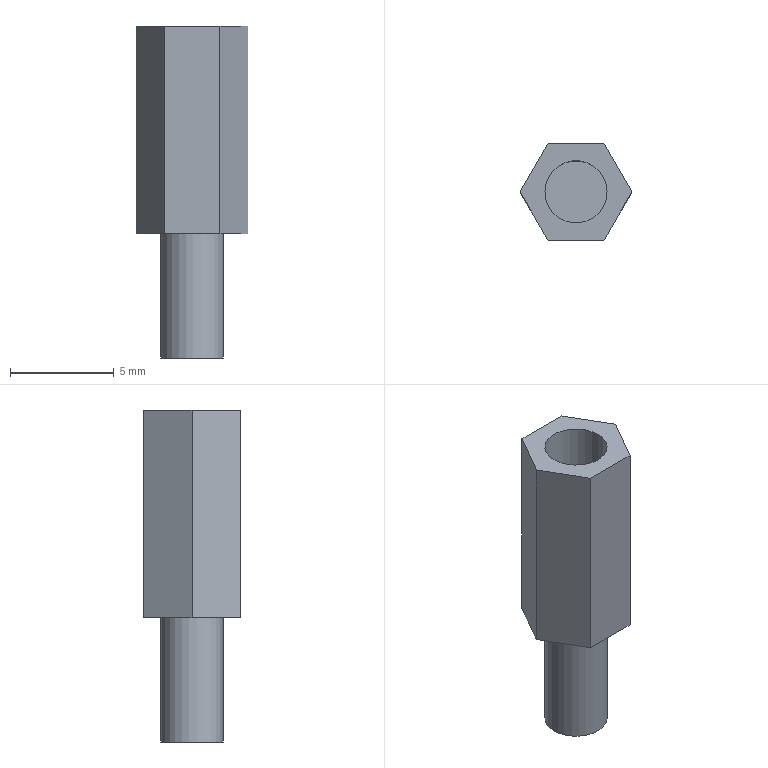Component | NX | M3_STANDOFF_2 | 1 solid | 12 faces | box 5.39 x 4.67 x 16 mm | volume 202 mm3 | plane 10 | cylinder 2 | commonest cylinder face diameters 3 x2
STEP:
#1=CARTESIAN_POINT('',(0.,0.,0.));
#2=DIRECTION('',(0.,0.,1.));
#3=DIRECTION('',(1.,0.,0.));
#4=AXIS2_PLACEMENT_3D('',#1,#2,#3);
#5=CARTESIAN_POINT('',(-97.523,127.67,-5.38));
#6=VERTEX_POINT('',#5);
#7=CARTESIAN_POINT('',(-98.871,125.335,-5.38));
#8=VERTEX_POINT('',#7);
#9=CARTESIAN_POINT('',(-97.523,127.67,-5.38));
#10=DIRECTION('',(-0.5,-0.866,0.));
#11=VECTOR('',#10,1.);
#12=LINE('',#9,#11);
#13=CARTESIAN_POINT('',(-97.523,127.67,4.62));
#14=DIRECTION('',(0.866,-0.5,0.));
#15=DIRECTION('',(-0.5,-0.866,0.));
#16=AXIS2_PLACEMENT_3D('',#13,#14,#15);
#17=PLANE('',#16);
#18=CARTESIAN_POINT('',(0.,10.));
#19=DIRECTION('',(1.,0.));
#20=VECTOR('',#19,1.);
#21=LINE('',#18,#20);
#22=(GEOMETRIC_REPRESENTATION_CONTEXT(2)PARAMETRIC_REPRESENTATION_CONTEXT()REPRESENTATION_CONTEXT('',''));
#23=DEFINITIONAL_REPRESENTATION('',(#21),#22);
#24=PCURVE('',#17,#23);
#25=CARTESIAN_POINT('',(-100.219,127.67,-5.38));
#26=DIRECTION('',(0.,0.,-1.));
#27=DIRECTION('',(-1.,0.,0.));
#28=AXIS2_PLACEMENT_3D('',#25,#26,#27);
#29=PLANE('',#28);
#30=CARTESIAN_POINT('',(-2.696,0.));
#31=DIRECTION('',(0.5,-0.866));
#32=VECTOR('',#31,1.);
#33=LINE('',#30,#32);
#34=(GEOMETRIC_REPRESENTATION_CONTEXT(2)PARAMETRIC_REPRESENTATION_CONTEXT()REPRESENTATION_CONTEXT('',''));
#35=DEFINITIONAL_REPRESENTATION('',(#33),#34);
#36=PCURVE('',#29,#35);
#37=SURFACE_CURVE('',#12,(#24,#36),.PCURVE_S1.);
#38=EDGE_CURVE('',#6,#8,#37,.T.);
#39=ORIENTED_EDGE('',*,*,#38,.F.);
#40=CARTESIAN_POINT('',(-97.523,127.67,4.62));
#41=VERTEX_POINT('',#40);
#42=CARTESIAN_POINT('',(-97.523,127.67,4.62));
#43=DIRECTION('',(0.,0.,-1.));
#44=VECTOR('',#43,1.);
#45=LINE('',#42,#44);
#46=CARTESIAN_POINT('',(0.,0.));
#47=DIRECTION('',(0.,1.));
#48=VECTOR('',#47,1.);
#49=LINE('',#46,#48);
#50=(GEOMETRIC_REPRESENTATION_CONTEXT(2)PARAMETRIC_REPRESENTATION_CONTEXT()REPRESENTATION_CONTEXT('',''));
#51=DEFINITIONAL_REPRESENTATION('',(#49),#50);
#52=PCURVE('',#17,#51);
#53=CARTESIAN_POINT('',(-98.871,130.005,4.62));
#54=DIRECTION('',(0.866,0.5,0.));
#55=DIRECTION('',(0.5,-0.866,0.));
#56=AXIS2_PLACEMENT_3D('',#53,#54,#55);
#57=PLANE('',#56);
#58=CARTESIAN_POINT('',(2.696,0.));
#59=DIRECTION('',(0.,1.));
#60=VECTOR('',#59,1.);
#61=LINE('',#58,#60);
#62=(GEOMETRIC_REPRESENTATION_CONTEXT(2)PARAMETRIC_REPRESENTATION_CONTEXT()REPRESENTATION_CONTEXT('',''));
#63=DEFINITIONAL_REPRESENTATION('',(#61),#62);
#64=PCURVE('',#57,#63);
#65=SURFACE_CURVE('',#45,(#52,#64),.PCURVE_S1.);
#66=EDGE_CURVE('',#41,#6,#65,.T.);
#67=ORIENTED_EDGE('',*,*,#66,.F.);
#68=CARTESIAN_POINT('',(-98.871,125.335,4.62));
#69=VERTEX_POINT('',#68);
#70=CARTESIAN_POINT('',(-97.523,127.67,4.62));
#71=DIRECTION('',(-0.5,-0.866,0.));
#72=VECTOR('',#71,1.);
#73=LINE('',#70,#72);
#74=CARTESIAN_POINT('',(0.,0.));
#75=DIRECTION('',(1.,0.));
#76=VECTOR('',#75,1.);
#77=LINE('',#74,#76);
#78=(GEOMETRIC_REPRESENTATION_CONTEXT(2)PARAMETRIC_REPRESENTATION_CONTEXT()REPRESENTATION_CONTEXT('',''));
#79=DEFINITIONAL_REPRESENTATION('',(#77),#78);
#80=PCURVE('',#17,#79);
#81=CARTESIAN_POINT('',(-100.219,127.67,4.62));
#82=DIRECTION('',(0.,0.,-1.));
#83=DIRECTION('',(-1.,0.,0.));
#84=AXIS2_PLACEMENT_3D('',#81,#82,#83);
#85=PLANE('',#84);
#86=CARTESIAN_POINT('',(-2.696,0.));
#87=DIRECTION('',(0.5,-0.866));
#88=VECTOR('',#87,1.);
#89=LINE('',#86,#88);
#90=(GEOMETRIC_REPRESENTATION_CONTEXT(2)PARAMETRIC_REPRESENTATION_CONTEXT()REPRESENTATION_CONTEXT('',''));
#91=DEFINITIONAL_REPRESENTATION('',(#89),#90);
#92=PCURVE('',#85,#91);
#93=SURFACE_CURVE('',#73,(#80,#92),.PCURVE_S1.);
#94=EDGE_CURVE('',#41,#69,#93,.T.);
#95=ORIENTED_EDGE('',*,*,#94,.T.);
#96=CARTESIAN_POINT('',(-98.871,125.335,4.62));
#97=DIRECTION('',(0.,0.,-1.));
#98=VECTOR('',#97,1.);
#99=LINE('',#96,#98);
#100=CARTESIAN_POINT('',(2.696,0.));
#101=DIRECTION('',(0.,1.));
#102=VECTOR('',#101,1.);
#103=LINE('',#100,#102);
#104=(GEOMETRIC_REPRESENTATION_CONTEXT(2)PARAMETRIC_REPRESENTATION_CONTEXT()REPRESENTATION_CONTEXT('',''));
#105=DEFINITIONAL_REPRESENTATION('',(#103),#104);
#106=PCURVE('',#17,#105);
#107=CARTESIAN_POINT('',(-98.871,125.335,4.62));
#108=DIRECTION('',(0.,-1.,0.));
#109=DIRECTION('',(-1.,-0.,0.));
#110=AXIS2_PLACEMENT_3D('',#107,#108,#109);
#111=PLANE('',#110);
#112=CARTESIAN_POINT('',(0.,0.));
#113=DIRECTION('',(0.,1.));
#114=VECTOR('',#113,1.);
#115=LINE('',#112,#114);
#116=(GEOMETRIC_REPRESENTATION_CONTEXT(2)PARAMETRIC_REPRESENTATION_CONTEXT()REPRESENTATION_CONTEXT('',''));
#117=DEFINITIONAL_REPRESENTATION('',(#115),#116);
#118=PCURVE('',#111,#117);
#119=SURFACE_CURVE('',#99,(#106,#118),.PCURVE_S1.);
#120=EDGE_CURVE('',#69,#8,#119,.T.);
#121=ORIENTED_EDGE('',*,*,#120,.T.);
#122=EDGE_LOOP('',(#39,#67,#95,#121));
#123=FACE_BOUND('',#122,.T.);
#124=ADVANCED_FACE('',(#123),#17,.T.);
#125=CARTESIAN_POINT('',(-101.567,125.335,-5.38));
#126=VERTEX_POINT('',#125);
#127=CARTESIAN_POINT('',(-98.871,125.335,-5.38));
#128=DIRECTION('',(-1.,-0.,0.));
#129=VECTOR('',#128,1.);
#130=LINE('',#127,#129);
#131=CARTESIAN_POINT('',(0.,10.));
#132=DIRECTION('',(1.,0.));
#133=VECTOR('',#132,1.);
#134=LINE('',#131,#133);
#135=(GEOMETRIC_REPRESENTATION_CONTEXT(2)PARAMETRIC_REPRESENTATION_CONTEXT()REPRESENTATION_CONTEXT('',''));
#136=DEFINITIONAL_REPRESENTATION('',(#134),#135);
#137=PCURVE('',#111,#136);
#138=CARTESIAN_POINT('',(-1.348,-2.335));
#139=DIRECTION('',(1.,-0.));
#140=VECTOR('',#139,1.);
#141=LINE('',#138,#140);
#142=(GEOMETRIC_REPRESENTATION_CONTEXT(2)PARAMETRIC_REPRESENTATION_CONTEXT()REPRESENTATION_CONTEXT('',''));
#143=DEFINITIONAL_REPRESENTATION('',(#141),#142);
#144=PCURVE('',#29,#143);
#145=SURFACE_CURVE('',#130,(#137,#144),.PCURVE_S1.);
#146=EDGE_CURVE('',#8,#126,#145,.T.);
#147=ORIENTED_EDGE('',*,*,#146,.F.);
#148=ORIENTED_EDGE('',*,*,#120,.F.);
#149=CARTESIAN_POINT('',(-101.567,125.335,4.62));
#150=VERTEX_POINT('',#149);
#151=CARTESIAN_POINT('',(-98.871,125.335,4.62));
#152=DIRECTION('',(-1.,-0.,0.));
#153=VECTOR('',#152,1.);
#154=LINE('',#151,#153);
#155=CARTESIAN_POINT('',(0.,0.));
#156=DIRECTION('',(1.,0.));
#157=VECTOR('',#156,1.);
#158=LINE('',#155,#157);
#159=(GEOMETRIC_REPRESENTATION_CONTEXT(2)PARAMETRIC_REPRESENTATION_CONTEXT()REPRESENTATION_CONTEXT('',''));
#160=DEFINITIONAL_REPRESENTATION('',(#158),#159);
#161=PCURVE('',#111,#160);
#162=CARTESIAN_POINT('',(-1.348,-2.335));
#163=DIRECTION('',(1.,-0.));
#164=VECTOR('',#163,1.);
#165=LINE('',#162,#164);
#166=(GEOMETRIC_REPRESENTATION_CONTEXT(2)PARAMETRIC_REPRESENTATION_CONTEXT()REPRESENTATION_CONTEXT('',''));
#167=DEFINITIONAL_REPRESENTATION('',(#165),#166);
#168=PCURVE('',#85,#167);
#169=SURFACE_CURVE('',#154,(#161,#168),.PCURVE_S1.);
#170=EDGE_CURVE('',#69,#150,#169,.T.);
#171=ORIENTED_EDGE('',*,*,#170,.T.);
#172=CARTESIAN_POINT('',(-101.567,125.335,4.62));
#173=DIRECTION('',(0.,0.,-1.));
#174=VECTOR('',#173,1.);
#175=LINE('',#172,#174);
#176=CARTESIAN_POINT('',(2.696,0.));
#177=DIRECTION('',(0.,1.));
#178=VECTOR('',#177,1.);
#179=LINE('',#176,#178);
#180=(GEOMETRIC_REPRESENTATION_CONTEXT(2)PARAMETRIC_REPRESENTATION_CONTEXT()REPRESENTATION_CONTEXT('',''));
#181=DEFINITIONAL_REPRESENTATION('',(#179),#180);
#182=PCURVE('',#111,#181);
#183=CARTESIAN_POINT('',(-101.567,125.335,4.62));
#184=DIRECTION('',(-0.866,-0.5,0.));
#185=DIRECTION('',(-0.5,0.866,0.));
#186=AXIS2_PLACEMENT_3D('',#183,#184,#185);
#187=PLANE('',#186);
#188=CARTESIAN_POINT('',(0.,0.));
#189=DIRECTION('',(0.,1.));
#190=VECTOR('',#189,1.);
#191=LINE('',#188,#190);
#192=(GEOMETRIC_REPRESENTATION_CONTEXT(2)PARAMETRIC_REPRESENTATION_CONTEXT()REPRESENTATION_CONTEXT('',''));
#193=DEFINITIONAL_REPRESENTATION('',(#191),#192);
#194=PCURVE('',#187,#193);
#195=SURFACE_CURVE('',#175,(#182,#194),.PCURVE_S1.);
#196=EDGE_CURVE('',#150,#126,#195,.T.);
#197=ORIENTED_EDGE('',*,*,#196,.T.);
#198=EDGE_LOOP('',(#147,#148,#171,#197));
#199=FACE_BOUND('',#198,.T.);
#200=ADVANCED_FACE('',(#199),#111,.T.);
#201=CARTESIAN_POINT('',(-102.915,127.67,-5.38));
#202=VERTEX_POINT('',#201);
#203=CARTESIAN_POINT('',(-101.567,125.335,-5.38));
#204=DIRECTION('',(-0.5,0.866,0.));
#205=VECTOR('',#204,1.);
#206=LINE('',#203,#205);
#207=CARTESIAN_POINT('',(0.,10.));
#208=DIRECTION('',(1.,0.));
#209=VECTOR('',#208,1.);
#210=LINE('',#207,#209);
#211=(GEOMETRIC_REPRESENTATION_CONTEXT(2)PARAMETRIC_REPRESENTATION_CONTEXT()REPRESENTATION_CONTEXT('',''));
#212=DEFINITIONAL_REPRESENTATION('',(#210),#211);
#213=PCURVE('',#187,#212);
#214=CARTESIAN_POINT('',(1.348,-2.335));
#215=DIRECTION('',(0.5,0.866));
#216=VECTOR('',#215,1.);
#217=LINE('',#214,#216);
#218=(GEOMETRIC_REPRESENTATION_CONTEXT(2)PARAMETRIC_REPRESENTATION_CONTEXT()REPRESENTATION_CONTEXT('',''));
#219=DEFINITIONAL_REPRESENTATION('',(#217),#218);
#220=PCURVE('',#29,#219);
#221=SURFACE_CURVE('',#206,(#213,#220),.PCURVE_S1.);
#222=EDGE_CURVE('',#126,#202,#221,.T.);
#223=ORIENTED_EDGE('',*,*,#222,.F.);
#224=ORIENTED_EDGE('',*,*,#196,.F.);
#225=CARTESIAN_POINT('',(-102.915,127.67,4.62));
#226=VERTEX_POINT('',#225);
#227=CARTESIAN_POINT('',(-101.567,125.335,4.62));
#228=DIRECTION('',(-0.5,0.866,0.));
#229=VECTOR('',#228,1.);
#230=LINE('',#227,#229);
#231=CARTESIAN_POINT('',(0.,0.));
#232=DIRECTION('',(1.,0.));
#233=VECTOR('',#232,1.);
#234=LINE('',#231,#233);
#235=(GEOMETRIC_REPRESENTATION_CONTEXT(2)PARAMETRIC_REPRESENTATION_CONTEXT()REPRESENTATION_CONTEXT('',''));
#236=DEFINITIONAL_REPRESENTATION('',(#234),#235);
#237=PCURVE('',#187,#236);
#238=CARTESIAN_POINT('',(1.348,-2.335));
#239=DIRECTION('',(0.5,0.866));
#240=VECTOR('',#239,1.);
#241=LINE('',#238,#240);
#242=(GEOMETRIC_REPRESENTATION_CONTEXT(2)PARAMETRIC_REPRESENTATION_CONTEXT()REPRESENTATION_CONTEXT('',''));
#243=DEFINITIONAL_REPRESENTATION('',(#241),#242);
#244=PCURVE('',#85,#243);
#245=SURFACE_CURVE('',#230,(#237,#244),.PCURVE_S1.);
#246=EDGE_CURVE('',#150,#226,#245,.T.);
#247=ORIENTED_EDGE('',*,*,#246,.T.);
#248=CARTESIAN_POINT('',(-102.915,127.67,4.62));
#249=DIRECTION('',(0.,0.,-1.));
#250=VECTOR('',#249,1.);
#251=LINE('',#248,#250);
#252=CARTESIAN_POINT('',(2.696,0.));
#253=DIRECTION('',(0.,1.));
#254=VECTOR('',#253,1.);
#255=LINE('',#252,#254);
#256=(GEOMETRIC_REPRESENTATION_CONTEXT(2)PARAMETRIC_REPRESENTATION_CONTEXT()REPRESENTATION_CONTEXT('',''));
#257=DEFINITIONAL_REPRESENTATION('',(#255),#256);
#258=PCURVE('',#187,#257);
#259=CARTESIAN_POINT('',(-102.915,127.67,4.62));
#260=DIRECTION('',(-0.866,0.5,0.));
#261=DIRECTION('',(0.5,0.866,0.));
#262=AXIS2_PLACEMENT_3D('',#259,#260,#261);
#263=PLANE('',#262);
#264=CARTESIAN_POINT('',(0.,0.));
#265=DIRECTION('',(0.,1.));
#266=VECTOR('',#265,1.);
#267=LINE('',#264,#266);
#268=(GEOMETRIC_REPRESENTATION_CONTEXT(2)PARAMETRIC_REPRESENTATION_CONTEXT()REPRESENTATION_CONTEXT('',''));
#269=DEFINITIONAL_REPRESENTATION('',(#267),#268);
#270=PCURVE('',#263,#269);
#271=SURFACE_CURVE('',#251,(#258,#270),.PCURVE_S1.);
#272=EDGE_CURVE('',#226,#202,#271,.T.);
#273=ORIENTED_EDGE('',*,*,#272,.T.);
#274=EDGE_LOOP('',(#223,#224,#247,#273));
#275=FACE_BOUND('',#274,.T.);
#276=ADVANCED_FACE('',(#275),#187,.T.);
#277=CARTESIAN_POINT('',(-101.567,130.005,-5.38));
#278=VERTEX_POINT('',#277);
#279=CARTESIAN_POINT('',(-102.915,127.67,-5.38));
#280=DIRECTION('',(0.5,0.866,0.));
#281=VECTOR('',#280,1.);
#282=LINE('',#279,#281);
#283=CARTESIAN_POINT('',(0.,10.));
#284=DIRECTION('',(1.,0.));
#285=VECTOR('',#284,1.);
#286=LINE('',#283,#285);
#287=(GEOMETRIC_REPRESENTATION_CONTEXT(2)PARAMETRIC_REPRESENTATION_CONTEXT()REPRESENTATION_CONTEXT('',''));
#288=DEFINITIONAL_REPRESENTATION('',(#286),#287);
#289=PCURVE('',#263,#288);
#290=CARTESIAN_POINT('',(2.696,0.));
#291=DIRECTION('',(-0.5,0.866));
#292=VECTOR('',#291,1.);
#293=LINE('',#290,#292);
#294=(GEOMETRIC_REPRESENTATION_CONTEXT(2)PARAMETRIC_REPRESENTATION_CONTEXT()REPRESENTATION_CONTEXT('',''));
#295=DEFINITIONAL_REPRESENTATION('',(#293),#294);
#296=PCURVE('',#29,#295);
#297=SURFACE_CURVE('',#282,(#289,#296),.PCURVE_S1.);
#298=EDGE_CURVE('',#202,#278,#297,.T.);
#299=ORIENTED_EDGE('',*,*,#298,.F.);
#300=ORIENTED_EDGE('',*,*,#272,.F.);
#301=CARTESIAN_POINT('',(-101.567,130.005,4.62));
#302=VERTEX_POINT('',#301);
#303=CARTESIAN_POINT('',(-102.915,127.67,4.62));
#304=DIRECTION('',(0.5,0.866,0.));
#305=VECTOR('',#304,1.);
#306=LINE('',#303,#305);
#307=CARTESIAN_POINT('',(0.,0.));
#308=DIRECTION('',(1.,0.));
#309=VECTOR('',#308,1.);
#310=LINE('',#307,#309);
#311=(GEOMETRIC_REPRESENTATION_CONTEXT(2)PARAMETRIC_REPRESENTATION_CONTEXT()REPRESENTATION_CONTEXT('',''));
#312=DEFINITIONAL_REPRESENTATION('',(#310),#311);
#313=PCURVE('',#263,#312);
#314=CARTESIAN_POINT('',(2.696,0.));
#315=DIRECTION('',(-0.5,0.866));
#316=VECTOR('',#315,1.);
#317=LINE('',#314,#316);
#318=(GEOMETRIC_REPRESENTATION_CONTEXT(2)PARAMETRIC_REPRESENTATION_CONTEXT()REPRESENTATION_CONTEXT('',''));
#319=DEFINITIONAL_REPRESENTATION('',(#317),#318);
#320=PCURVE('',#85,#319);
#321=SURFACE_CURVE('',#306,(#313,#320),.PCURVE_S1.);
#322=EDGE_CURVE('',#226,#302,#321,.T.);
#323=ORIENTED_EDGE('',*,*,#322,.T.);
#324=CARTESIAN_POINT('',(-101.567,130.005,4.62));
#325=DIRECTION('',(0.,0.,-1.));
#326=VECTOR('',#325,1.);
#327=LINE('',#324,#326);
#328=CARTESIAN_POINT('',(2.696,0.));
#329=DIRECTION('',(0.,1.));
#330=VECTOR('',#329,1.);
#331=LINE('',#328,#330);
#332=(GEOMETRIC_REPRESENTATION_CONTEXT(2)PARAMETRIC_REPRESENTATION_CONTEXT()REPRESENTATION_CONTEXT('',''));
#333=DEFINITIONAL_REPRESENTATION('',(#331),#332);
#334=PCURVE('',#263,#333);
#335=CARTESIAN_POINT('',(-101.567,130.005,4.62));
#336=DIRECTION('',(-0.,1.,0.));
#337=DIRECTION('',(1.,0.,0.));
#338=AXIS2_PLACEMENT_3D('',#335,#336,#337);
#339=PLANE('',#338);
#340=CARTESIAN_POINT('',(0.,0.));
#341=DIRECTION('',(0.,1.));
#342=VECTOR('',#341,1.);
#343=LINE('',#340,#342);
#344=(GEOMETRIC_REPRESENTATION_CONTEXT(2)PARAMETRIC_REPRESENTATION_CONTEXT()REPRESENTATION_CONTEXT('',''));
#345=DEFINITIONAL_REPRESENTATION('',(#343),#344);
#346=PCURVE('',#339,#345);
#347=SURFACE_CURVE('',#327,(#334,#346),.PCURVE_S1.);
#348=EDGE_CURVE('',#302,#278,#347,.T.);
#349=ORIENTED_EDGE('',*,*,#348,.T.);
#350=EDGE_LOOP('',(#299,#300,#323,#349));
#351=FACE_BOUND('',#350,.T.);
#352=ADVANCED_FACE('',(#351),#263,.T.);
#353=CARTESIAN_POINT('',(-98.871,130.005,-5.38));
#354=VERTEX_POINT('',#353);
#355=CARTESIAN_POINT('',(-101.567,130.005,-5.38));
#356=DIRECTION('',(1.,0.,0.));
#357=VECTOR('',#356,1.);
#358=LINE('',#355,#357);
#359=CARTESIAN_POINT('',(0.,10.));
#360=DIRECTION('',(1.,0.));
#361=VECTOR('',#360,1.);
#362=LINE('',#359,#361);
#363=(GEOMETRIC_REPRESENTATION_CONTEXT(2)PARAMETRIC_REPRESENTATION_CONTEXT()REPRESENTATION_CONTEXT('',''));
#364=DEFINITIONAL_REPRESENTATION('',(#362),#363);
#365=PCURVE('',#339,#364);
#366=CARTESIAN_POINT('',(1.348,2.335));
#367=DIRECTION('',(-1.,0.));
#368=VECTOR('',#367,1.);
#369=LINE('',#366,#368);
#370=(GEOMETRIC_REPRESENTATION_CONTEXT(2)PARAMETRIC_REPRESENTATION_CONTEXT()REPRESENTATION_CONTEXT('',''));
#371=DEFINITIONAL_REPRESENTATION('',(#369),#370);
#372=PCURVE('',#29,#371);
#373=SURFACE_CURVE('',#358,(#365,#372),.PCURVE_S1.);
#374=EDGE_CURVE('',#278,#354,#373,.T.);
#375=ORIENTED_EDGE('',*,*,#374,.F.);
#376=ORIENTED_EDGE('',*,*,#348,.F.);
#377=CARTESIAN_POINT('',(-98.871,130.005,4.62));
#378=VERTEX_POINT('',#377);
#379=CARTESIAN_POINT('',(-101.567,130.005,4.62));
#380=DIRECTION('',(1.,0.,0.));
#381=VECTOR('',#380,1.);
#382=LINE('',#379,#381);
#383=CARTESIAN_POINT('',(0.,0.));
#384=DIRECTION('',(1.,0.));
#385=VECTOR('',#384,1.);
#386=LINE('',#383,#385);
#387=(GEOMETRIC_REPRESENTATION_CONTEXT(2)PARAMETRIC_REPRESENTATION_CONTEXT()REPRESENTATION_CONTEXT('',''));
#388=DEFINITIONAL_REPRESENTATION('',(#386),#387);
#389=PCURVE('',#339,#388);
#390=CARTESIAN_POINT('',(1.348,2.335));
#391=DIRECTION('',(-1.,0.));
#392=VECTOR('',#391,1.);
#393=LINE('',#390,#392);
#394=(GEOMETRIC_REPRESENTATION_CONTEXT(2)PARAMETRIC_REPRESENTATION_CONTEXT()REPRESENTATION_CONTEXT('',''));
#395=DEFINITIONAL_REPRESENTATION('',(#393),#394);
#396=PCURVE('',#85,#395);
#397=SURFACE_CURVE('',#382,(#389,#396),.PCURVE_S1.);
#398=EDGE_CURVE('',#302,#378,#397,.T.);
#399=ORIENTED_EDGE('',*,*,#398,.T.);
#400=CARTESIAN_POINT('',(-98.871,130.005,4.62));
#401=DIRECTION('',(0.,0.,-1.));
#402=VECTOR('',#401,1.);
#403=LINE('',#400,#402);
#404=CARTESIAN_POINT('',(2.696,0.));
#405=DIRECTION('',(0.,1.));
#406=VECTOR('',#405,1.);
#407=LINE('',#404,#406);
#408=(GEOMETRIC_REPRESENTATION_CONTEXT(2)PARAMETRIC_REPRESENTATION_CONTEXT()REPRESENTATION_CONTEXT('',''));
#409=DEFINITIONAL_REPRESENTATION('',(#407),#408);
#410=PCURVE('',#339,#409);
#411=CARTESIAN_POINT('',(0.,0.));
#412=DIRECTION('',(0.,1.));
#413=VECTOR('',#412,1.);
#414=LINE('',#411,#413);
#415=(GEOMETRIC_REPRESENTATION_CONTEXT(2)PARAMETRIC_REPRESENTATION_CONTEXT()REPRESENTATION_CONTEXT('',''));
#416=DEFINITIONAL_REPRESENTATION('',(#414),#415);
#417=PCURVE('',#57,#416);
#418=SURFACE_CURVE('',#403,(#410,#417),.PCURVE_S1.);
#419=EDGE_CURVE('',#378,#354,#418,.T.);
#420=ORIENTED_EDGE('',*,*,#419,.T.);
#421=EDGE_LOOP('',(#375,#376,#399,#420));
#422=FACE_BOUND('',#421,.T.);
#423=ADVANCED_FACE('',(#422),#339,.T.);
#424=CARTESIAN_POINT('',(-98.871,130.005,-5.38));
#425=DIRECTION('',(0.5,-0.866,0.));
#426=VECTOR('',#425,1.);
#427=LINE('',#424,#426);
#428=CARTESIAN_POINT('',(0.,10.));
#429=DIRECTION('',(1.,0.));
#430=VECTOR('',#429,1.);
#431=LINE('',#428,#430);
#432=(GEOMETRIC_REPRESENTATION_CONTEXT(2)PARAMETRIC_REPRESENTATION_CONTEXT()REPRESENTATION_CONTEXT('',''));
#433=DEFINITIONAL_REPRESENTATION('',(#431),#432);
#434=PCURVE('',#57,#433);
#435=CARTESIAN_POINT('',(-1.348,2.335));
#436=DIRECTION('',(-0.5,-0.866));
#437=VECTOR('',#436,1.);
#438=LINE('',#435,#437);
#439=(GEOMETRIC_REPRESENTATION_CONTEXT(2)PARAMETRIC_REPRESENTATION_CONTEXT()REPRESENTATION_CONTEXT('',''));
#440=DEFINITIONAL_REPRESENTATION('',(#438),#439);
#441=PCURVE('',#29,#440);
#442=SURFACE_CURVE('',#427,(#434,#441),.PCURVE_S1.);
#443=EDGE_CURVE('',#354,#6,#442,.T.);
#444=ORIENTED_EDGE('',*,*,#443,.F.);
#445=ORIENTED_EDGE('',*,*,#419,.F.);
#446=CARTESIAN_POINT('',(-98.871,130.005,4.62));
#447=DIRECTION('',(0.5,-0.866,0.));
#448=VECTOR('',#447,1.);
#449=LINE('',#446,#448);
#450=CARTESIAN_POINT('',(0.,0.));
#451=DIRECTION('',(1.,0.));
#452=VECTOR('',#451,1.);
#453=LINE('',#450,#452);
#454=(GEOMETRIC_REPRESENTATION_CONTEXT(2)PARAMETRIC_REPRESENTATION_CONTEXT()REPRESENTATION_CONTEXT('',''));
#455=DEFINITIONAL_REPRESENTATION('',(#453),#454);
#456=PCURVE('',#57,#455);
#457=CARTESIAN_POINT('',(-1.348,2.335));
#458=DIRECTION('',(-0.5,-0.866));
#459=VECTOR('',#458,1.);
#460=LINE('',#457,#459);
#461=(GEOMETRIC_REPRESENTATION_CONTEXT(2)PARAMETRIC_REPRESENTATION_CONTEXT()REPRESENTATION_CONTEXT('',''));
#462=DEFINITIONAL_REPRESENTATION('',(#460),#461);
#463=PCURVE('',#85,#462);
#464=SURFACE_CURVE('',#449,(#456,#463),.PCURVE_S1.);
#465=EDGE_CURVE('',#378,#41,#464,.T.);
#466=ORIENTED_EDGE('',*,*,#465,.T.);
#467=ORIENTED_EDGE('',*,*,#66,.T.);
#468=EDGE_LOOP('',(#444,#445,#466,#467));
#469=FACE_BOUND('',#468,.T.);
#470=ADVANCED_FACE('',(#469),#57,.T.);
#471=CARTESIAN_POINT('',(-98.719,127.67,4.62));
#472=VERTEX_POINT('',#471);
#473=CARTESIAN_POINT('',(-100.219,127.67,4.62));
#474=DIRECTION('',(0.,0.,-1.));
#475=DIRECTION('',(1.,0.,0.));
#476=AXIS2_PLACEMENT_3D('',#473,#474,#475);
#477=CIRCLE('',#476,1.5);
#478=CARTESIAN_POINT('',(0.,0.));
#479=DIRECTION('',(-1.,0.));
#480=AXIS2_PLACEMENT_2D('',#478,#479);
#481=CIRCLE('',#480,1.5);
#482=(GEOMETRIC_REPRESENTATION_CONTEXT(2)PARAMETRIC_REPRESENTATION_CONTEXT()REPRESENTATION_CONTEXT('',''));
#483=DEFINITIONAL_REPRESENTATION('',(#481),#482);
#484=PCURVE('',#85,#483);
#485=CARTESIAN_POINT('',(-100.219,127.67,4.62));
#486=DIRECTION('',(0.,0.,-1.));
#487=DIRECTION('',(-1.,0.,0.));
#488=AXIS2_PLACEMENT_3D('',#485,#486,#487);
#489=CYLINDRICAL_SURFACE('',#488,1.5);
#490=CARTESIAN_POINT('',(3.142,0.));
#491=DIRECTION('',(1.,0.));
#492=VECTOR('',#491,1.);
#493=LINE('',#490,#492);
#494=(GEOMETRIC_REPRESENTATION_CONTEXT(2)PARAMETRIC_REPRESENTATION_CONTEXT()REPRESENTATION_CONTEXT('',''));
#495=DEFINITIONAL_REPRESENTATION('',(#493),#494);
#496=PCURVE('',#489,#495);
#497=SURFACE_CURVE('',#477,(#484,#496),.PCURVE_S1.);
#498=EDGE_CURVE('',#472,#472,#497,.T.);
#499=ORIENTED_EDGE('',*,*,#498,.T.);
#500=EDGE_LOOP('',(#499));
#501=FACE_BOUND('',#500,.T.);
#502=ORIENTED_EDGE('',*,*,#94,.F.);
#503=ORIENTED_EDGE('',*,*,#465,.F.);
#504=ORIENTED_EDGE('',*,*,#398,.F.);
#505=ORIENTED_EDGE('',*,*,#322,.F.);
#506=ORIENTED_EDGE('',*,*,#246,.F.);
#507=ORIENTED_EDGE('',*,*,#170,.F.);
#508=EDGE_LOOP('',(#502,#503,#504,#505,#506,#507));
#509=FACE_BOUND('',#508,.T.);
#510=ADVANCED_FACE('',(#501,#509),#85,.F.);
#511=CARTESIAN_POINT('',(-100.969,128.969,-5.38));
#512=VERTEX_POINT('',#511);
#513=CARTESIAN_POINT('',(-100.219,127.67,-5.38));
#514=DIRECTION('',(0.,0.,-1.));
#515=DIRECTION('',(-0.5,0.866,0.));
#516=AXIS2_PLACEMENT_3D('',#513,#514,#515);
#517=CIRCLE('',#516,1.5);
#518=CARTESIAN_POINT('',(0.,0.));
#519=DIRECTION('',(0.5,0.866));
#520=AXIS2_PLACEMENT_2D('',#518,#519);
#521=CIRCLE('',#520,1.5);
#522=(GEOMETRIC_REPRESENTATION_CONTEXT(2)PARAMETRIC_REPRESENTATION_CONTEXT()REPRESENTATION_CONTEXT('',''));
#523=DEFINITIONAL_REPRESENTATION('',(#521),#522);
#524=PCURVE('',#29,#523);
#525=CARTESIAN_POINT('',(-100.219,127.67,-5.38));
#526=DIRECTION('',(0.,0.,-1.));
#527=DIRECTION('',(-1.,0.,0.));
#528=AXIS2_PLACEMENT_3D('',#525,#526,#527);
#529=CYLINDRICAL_SURFACE('',#528,1.5);
#530=CARTESIAN_POINT('',(1.047,0.));
#531=DIRECTION('',(1.,0.));
#532=VECTOR('',#531,1.);
#533=LINE('',#530,#532);
#534=(GEOMETRIC_REPRESENTATION_CONTEXT(2)PARAMETRIC_REPRESENTATION_CONTEXT()REPRESENTATION_CONTEXT('',''));
#535=DEFINITIONAL_REPRESENTATION('',(#533),#534);
#536=PCURVE('',#529,#535);
#537=SURFACE_CURVE('',#517,(#524,#536),.PCURVE_S1.);
#538=EDGE_CURVE('',#512,#512,#537,.T.);
#539=ORIENTED_EDGE('',*,*,#538,.F.);
#540=EDGE_LOOP('',(#539));
#541=FACE_BOUND('',#540,.T.);
#542=ORIENTED_EDGE('',*,*,#38,.T.);
#543=ORIENTED_EDGE('',*,*,#146,.T.);
#544=ORIENTED_EDGE('',*,*,#222,.T.);
#545=ORIENTED_EDGE('',*,*,#298,.T.);
#546=ORIENTED_EDGE('',*,*,#374,.T.);
#547=ORIENTED_EDGE('',*,*,#443,.T.);
#548=EDGE_LOOP('',(#542,#543,#544,#545,#546,#547));
#549=FACE_BOUND('',#548,.T.);
#550=ADVANCED_FACE('',(#541,#549),#29,.T.);
#551=ORIENTED_EDGE('',*,*,#538,.T.);
#552=CARTESIAN_POINT('',(-100.969,128.969,-11.38));
#553=VERTEX_POINT('',#552);
#554=CARTESIAN_POINT('',(-100.969,128.969,-5.38));
#555=CARTESIAN_POINT('',(-100.969,128.969,-11.38));
#556=B_SPLINE_CURVE_WITH_KNOTS('',1,(#554,#555),.UNSPECIFIED.,.F.,.F.,(2,2),(0.,6.),.PIECEWISE_BEZIER_KNOTS.);
#557=CARTESIAN_POINT('',(7.33,0.));
#558=DIRECTION('',(0.,1.));
#559=VECTOR('',#558,1.);
#560=LINE('',#557,#559);
#561=(GEOMETRIC_REPRESENTATION_CONTEXT(2)PARAMETRIC_REPRESENTATION_CONTEXT()REPRESENTATION_CONTEXT('',''));
#562=DEFINITIONAL_REPRESENTATION('',(#560),#561);
#563=PCURVE('',#529,#562);
#564=CARTESIAN_POINT('',(1.047,0.));
#565=DIRECTION('',(0.,1.));
#566=VECTOR('',#565,1.);
#567=LINE('',#564,#566);
#568=(GEOMETRIC_REPRESENTATION_CONTEXT(2)PARAMETRIC_REPRESENTATION_CONTEXT()REPRESENTATION_CONTEXT('',''));
#569=DEFINITIONAL_REPRESENTATION('',(#567),#568);
#570=PCURVE('',#529,#569);
#571=SEAM_CURVE('',#556,(#563,#570),.PCURVE_S1.);
#572=EDGE_CURVE('',#512,#553,#571,.T.);
#573=ORIENTED_EDGE('',*,*,#572,.T.);
#574=CARTESIAN_POINT('',(-100.219,127.67,-11.38));
#575=DIRECTION('',(0.,0.,-1.));
#576=DIRECTION('',(-0.5,0.866,0.));
#577=AXIS2_PLACEMENT_3D('',#574,#575,#576);
#578=CIRCLE('',#577,1.5);
#579=CARTESIAN_POINT('',(1.047,6.));
#580=DIRECTION('',(1.,0.));
#581=VECTOR('',#580,1.);
#582=LINE('',#579,#581);
#583=(GEOMETRIC_REPRESENTATION_CONTEXT(2)PARAMETRIC_REPRESENTATION_CONTEXT()REPRESENTATION_CONTEXT('',''));
#584=DEFINITIONAL_REPRESENTATION('',(#582),#583);
#585=PCURVE('',#529,#584);
#586=CARTESIAN_POINT('',(-100.219,127.67,-11.38));
#587=DIRECTION('',(0.,0.,-1.));
#588=DIRECTION('',(-1.,0.,0.));
#589=AXIS2_PLACEMENT_3D('',#586,#587,#588);
#590=PLANE('',#589);
#591=CARTESIAN_POINT('',(0.,0.));
#592=DIRECTION('',(0.5,0.866));
#593=AXIS2_PLACEMENT_2D('',#591,#592);
#594=CIRCLE('',#593,1.5);
#595=(GEOMETRIC_REPRESENTATION_CONTEXT(2)PARAMETRIC_REPRESENTATION_CONTEXT()REPRESENTATION_CONTEXT('',''));
#596=DEFINITIONAL_REPRESENTATION('',(#594),#595);
#597=PCURVE('',#590,#596);
#598=SURFACE_CURVE('',#578,(#585,#597),.PCURVE_S1.);
#599=EDGE_CURVE('',#553,#553,#598,.T.);
#600=ORIENTED_EDGE('',*,*,#599,.F.);
#601=ORIENTED_EDGE('',*,*,#572,.F.);
#602=EDGE_LOOP('',(#551,#573,#600,#601));
#603=FACE_BOUND('',#602,.T.);
#604=ADVANCED_FACE('',(#603),#529,.T.);
#605=ORIENTED_EDGE('',*,*,#599,.T.);
#606=EDGE_LOOP('',(#605));
#607=FACE_BOUND('',#606,.T.);
#608=ADVANCED_FACE('',(#607),#590,.T.);
#609=ORIENTED_EDGE('',*,*,#498,.T.);
#610=CARTESIAN_POINT('',(-98.719,127.67,0.5199));
#611=VERTEX_POINT('',#610);
#612=CARTESIAN_POINT('',(-98.719,127.67,4.62));
#613=CARTESIAN_POINT('',(-98.719,127.67,0.5199));
#614=B_SPLINE_CURVE_WITH_KNOTS('',1,(#612,#613),.UNSPECIFIED.,.F.,.F.,(2,2),(0.,4.1),.PIECEWISE_BEZIER_KNOTS.);
#615=CARTESIAN_POINT('',(9.425,0.));
#616=DIRECTION('',(0.,1.));
#617=VECTOR('',#616,1.);
#618=LINE('',#615,#617);
#619=(GEOMETRIC_REPRESENTATION_CONTEXT(2)PARAMETRIC_REPRESENTATION_CONTEXT()REPRESENTATION_CONTEXT('',''));
#620=DEFINITIONAL_REPRESENTATION('',(#618),#619);
#621=PCURVE('',#489,#620);
#622=CARTESIAN_POINT('',(3.142,0.));
#623=DIRECTION('',(0.,1.));
#624=VECTOR('',#623,1.);
#625=LINE('',#622,#624);
#626=(GEOMETRIC_REPRESENTATION_CONTEXT(2)PARAMETRIC_REPRESENTATION_CONTEXT()REPRESENTATION_CONTEXT('',''));
#627=DEFINITIONAL_REPRESENTATION('',(#625),#626);
#628=PCURVE('',#489,#627);
#629=SEAM_CURVE('',#614,(#621,#628),.PCURVE_S1.);
#630=EDGE_CURVE('',#472,#611,#629,.T.);
#631=ORIENTED_EDGE('',*,*,#630,.T.);
#632=CARTESIAN_POINT('',(-100.219,127.67,0.5199));
#633=DIRECTION('',(0.,0.,1.));
#634=DIRECTION('',(1.,0.,0.));
#635=AXIS2_PLACEMENT_3D('',#632,#633,#634);
#636=CIRCLE('',#635,1.5);
#637=CARTESIAN_POINT('',(9.425,4.1));
#638=DIRECTION('',(-1.,0.));
#639=VECTOR('',#638,1.);
#640=LINE('',#637,#639);
#641=(GEOMETRIC_REPRESENTATION_CONTEXT(2)PARAMETRIC_REPRESENTATION_CONTEXT()REPRESENTATION_CONTEXT('',''));
#642=DEFINITIONAL_REPRESENTATION('',(#640),#641);
#643=PCURVE('',#489,#642);
#644=CARTESIAN_POINT('',(-100.219,127.67,0.5199));
#645=DIRECTION('',(0.,0.,-1.));
#646=DIRECTION('',(-1.,0.,0.));
#647=AXIS2_PLACEMENT_3D('',#644,#645,#646);
#648=PLANE('',#647);
#649=CARTESIAN_POINT('',(-1.5,0.));
#650=CARTESIAN_POINT('',(-1.5,2.598));
#651=CARTESIAN_POINT('',(0.75,1.299));
#652=CARTESIAN_POINT('',(3.,0.));
#653=CARTESIAN_POINT('',(0.75,-1.299));
#654=CARTESIAN_POINT('',(-1.5,-2.598));
#655=CARTESIAN_POINT('',(-1.5,0.));
#656=(BOUNDED_CURVE()B_SPLINE_CURVE(2,(#649,#650,#651,#652,#653,#654,#655),.UNSPECIFIED.,.T.,.F.)B_SPLINE_CURVE_WITH_KNOTS((1,2,2,2,2,1),(-2.094,0.,2.094,4.189,6.283,8.378),.UNSPECIFIED.)CURVE()GEOMETRIC_REPRESENTATION_ITEM()RATIONAL_B_SPLINE_CURVE((1.,0.5,1.,0.5,1.,0.5,1.))REPRESENTATION_ITEM(''));
#657=(GEOMETRIC_REPRESENTATION_CONTEXT(2)PARAMETRIC_REPRESENTATION_CONTEXT()REPRESENTATION_CONTEXT('',''));
#658=DEFINITIONAL_REPRESENTATION('',(#656),#657);
#659=PCURVE('',#648,#658);
#660=SURFACE_CURVE('',#636,(#643,#659),.PCURVE_S1.);
#661=EDGE_CURVE('',#611,#611,#660,.T.);
#662=ORIENTED_EDGE('',*,*,#661,.T.);
#663=ORIENTED_EDGE('',*,*,#630,.F.);
#664=EDGE_LOOP('',(#609,#631,#662,#663));
#665=FACE_BOUND('',#664,.F.);
#666=ADVANCED_FACE('',(#665),#489,.F.);
#667=ORIENTED_EDGE('',*,*,#661,.T.);
#668=EDGE_LOOP('',(#667));
#669=FACE_BOUND('',#668,.T.);
#670=ADVANCED_FACE('',(#669),#648,.F.);
#671=CLOSED_SHELL('',(#124,#200,#276,#352,#423,#470,#510,#550,#604,#608,#666,#670));
#672=MANIFOLD_SOLID_BREP('',#671);
#673=(LENGTH_UNIT()NAMED_UNIT(*)SI_UNIT(.MILLI.,.METRE.));
#674=UNCERTAINTY_MEASURE_WITH_UNIT(LENGTH_MEASURE(0.000002),#673,'','');
#675=(NAMED_UNIT(*)PLANE_ANGLE_UNIT()SI_UNIT($,.RADIAN.));
#676=(NAMED_UNIT(*)SI_UNIT($,.STERADIAN.)SOLID_ANGLE_UNIT());
#677=(GEOMETRIC_REPRESENTATION_CONTEXT(3)GLOBAL_UNCERTAINTY_ASSIGNED_CONTEXT((#674))GLOBAL_UNIT_ASSIGNED_CONTEXT((#673,#675,#676))REPRESENTATION_CONTEXT('',''));
#678=ADVANCED_BREP_SHAPE_REPRESENTATION('',(#4,#672),#677);